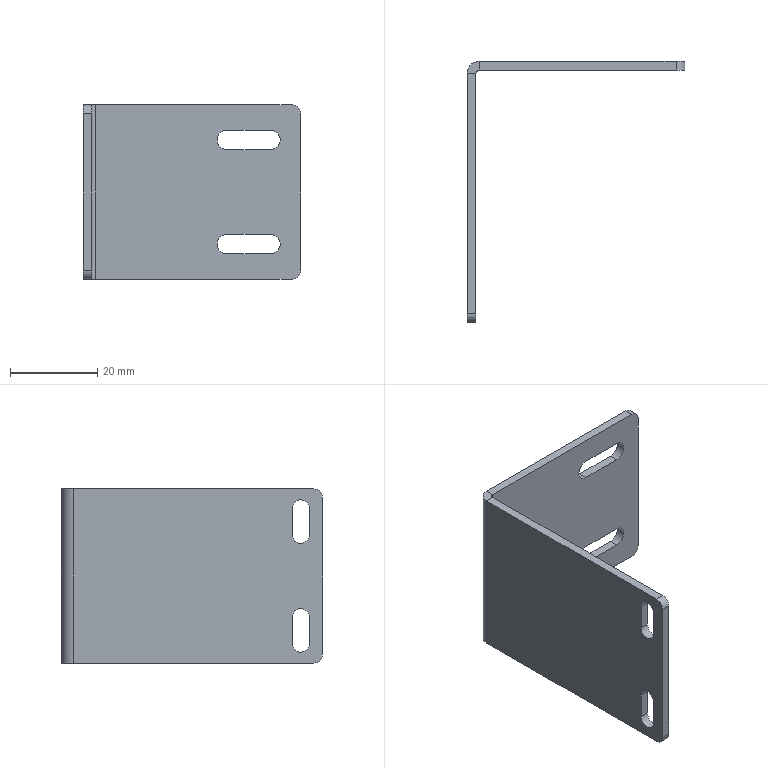Component | SolidWorks | MaterialDetectionSensorMountingPlate-2 | 1 solid | 34 faces | box 50 x 60 x 40 mm | volume 8184 mm3 | plane 20 | cylinder 14 | commonest cylinder face diameters 4 x8 4.5 x4 1.473 x1 5.473 x1
STEP:
#1=COLOUR_RGB('',0.7922,0.8196,0.9333);
#2=FILL_AREA_STYLE_COLOUR('',#1);
#3=FILL_AREA_STYLE('',(#2));
#4=SURFACE_STYLE_FILL_AREA(#3);
#5=SURFACE_SIDE_STYLE('',(#4));
#6=SURFACE_STYLE_USAGE(.BOTH.,#5);
#7=PRESENTATION_STYLE_ASSIGNMENT((#6));
#8=CARTESIAN_POINT('',(-8.239,51.713,4.331));
#9=VERTEX_POINT('',#8);
#10=CARTESIAN_POINT('',(-8.239,51.634,4.331));
#11=VERTEX_POINT('',#10);
#12=CARTESIAN_POINT('',(-8.239,51.713,4.331));
#13=DIRECTION('',(0.,-1.,0.));
#14=VECTOR('',#13,39.37);
#15=LINE('',#12,#14);
#16=EDGE_CURVE('',#9,#11,#15,.T.);
#17=ORIENTED_EDGE('',*,*,#16,.F.);
#18=CARTESIAN_POINT('',(-8.346,51.605,4.331));
#19=VERTEX_POINT('',#18);
#20=CARTESIAN_POINT('',(-8.239,51.605,4.331));
#21=DIRECTION('',(0.,0.,1.));
#22=DIRECTION('',(-1.,0.,0.));
#23=AXIS2_PLACEMENT_3D('',#20,#21,#22);
#24=CIRCLE('',#23,0.1077);
#25=EDGE_CURVE('',#9,#19,#24,.T.);
#26=ORIENTED_EDGE('',*,*,#25,.T.);
#27=CARTESIAN_POINT('',(-8.268,51.605,4.331));
#28=VERTEX_POINT('',#27);
#29=CARTESIAN_POINT('',(-8.268,51.605,4.331));
#30=DIRECTION('',(-1.,-0.,0.));
#31=VECTOR('',#30,39.37);
#32=LINE('',#29,#31);
#33=EDGE_CURVE('',#28,#19,#32,.T.);
#34=ORIENTED_EDGE('',*,*,#33,.F.);
#35=CARTESIAN_POINT('',(-8.239,51.605,4.331));
#36=DIRECTION('',(0.,0.,1.));
#37=DIRECTION('',(1.,0.,0.));
#38=AXIS2_PLACEMENT_3D('',#35,#36,#37);
#39=CIRCLE('',#38,0.029);
#40=EDGE_CURVE('',#11,#28,#39,.T.);
#41=ORIENTED_EDGE('',*,*,#40,.F.);
#42=EDGE_LOOP('',(#17,#26,#34,#41));
#43=FACE_OUTER_BOUND('',#42,.T.);
#44=CARTESIAN_POINT('',(-8.239,51.713,4.331));
#45=DIRECTION('',(0.,0.,1.));
#46=DIRECTION('',(1.,0.,0.));
#47=AXIS2_PLACEMENT_3D('',#44,#45,#46);
#48=PLANE('',#47);
#49=ADVANCED_FACE('',(#43),#48,.T.);
#50=CARTESIAN_POINT('',(-6.457,51.634,4.331));
#51=VERTEX_POINT('',#50);
#52=CARTESIAN_POINT('',(-8.346,51.634,4.331));
#53=DIRECTION('',(-1.,0.,0.));
#54=VECTOR('',#53,39.37);
#55=LINE('',#52,#54);
#56=EDGE_CURVE('',#51,#11,#55,.T.);
#57=ORIENTED_EDGE('',*,*,#56,.F.);
#58=CARTESIAN_POINT('',(-6.457,51.713,4.331));
#59=VERTEX_POINT('',#58);
#60=CARTESIAN_POINT('',(-6.457,51.605,4.331));
#61=DIRECTION('',(0.,1.,0.));
#62=VECTOR('',#61,39.37);
#63=LINE('',#60,#62);
#64=EDGE_CURVE('',#51,#59,#63,.T.);
#65=ORIENTED_EDGE('',*,*,#64,.T.);
#66=CARTESIAN_POINT('',(-8.346,51.713,4.331));
#67=DIRECTION('',(-1.,0.,0.));
#68=VECTOR('',#67,39.37);
#69=LINE('',#66,#68);
#70=EDGE_CURVE('',#59,#9,#69,.T.);
#71=ORIENTED_EDGE('',*,*,#70,.T.);
#72=ORIENTED_EDGE('',*,*,#16,.T.);
#73=EDGE_LOOP('',(#57,#65,#71,#72));
#74=FACE_OUTER_BOUND('',#73,.T.);
#75=CARTESIAN_POINT('',(-8.268,51.605,4.331));
#76=DIRECTION('',(0.,0.,1.));
#77=DIRECTION('',(1.,0.,0.));
#78=AXIS2_PLACEMENT_3D('',#75,#76,#77);
#79=PLANE('',#78);
#80=ADVANCED_FACE('',(#74),#79,.T.);
#81=CARTESIAN_POINT('',(-8.346,51.605,2.756));
#82=VERTEX_POINT('',#81);
#83=CARTESIAN_POINT('',(-8.268,51.605,2.756));
#84=VERTEX_POINT('',#83);
#85=CARTESIAN_POINT('',(-8.346,51.605,2.756));
#86=DIRECTION('',(1.,0.,0.));
#87=VECTOR('',#86,39.37);
#88=LINE('',#85,#87);
#89=EDGE_CURVE('',#82,#84,#88,.T.);
#90=ORIENTED_EDGE('',*,*,#89,.F.);
#91=CARTESIAN_POINT('',(-8.239,51.713,2.756));
#92=VERTEX_POINT('',#91);
#93=CARTESIAN_POINT('',(-8.239,51.605,2.756));
#94=DIRECTION('',(0.,0.,1.));
#95=DIRECTION('',(-1.,0.,0.));
#96=AXIS2_PLACEMENT_3D('',#93,#94,#95);
#97=CIRCLE('',#96,0.1077);
#98=EDGE_CURVE('',#92,#82,#97,.T.);
#99=ORIENTED_EDGE('',*,*,#98,.F.);
#100=CARTESIAN_POINT('',(-8.239,51.634,2.756));
#101=VERTEX_POINT('',#100);
#102=CARTESIAN_POINT('',(-8.239,51.634,2.756));
#103=DIRECTION('',(0.,1.,0.));
#104=VECTOR('',#103,39.37);
#105=LINE('',#102,#104);
#106=EDGE_CURVE('',#101,#92,#105,.T.);
#107=ORIENTED_EDGE('',*,*,#106,.F.);
#108=CARTESIAN_POINT('',(-8.239,51.605,2.756));
#109=DIRECTION('',(0.,0.,1.));
#110=DIRECTION('',(1.,0.,0.));
#111=AXIS2_PLACEMENT_3D('',#108,#109,#110);
#112=CIRCLE('',#111,0.029);
#113=EDGE_CURVE('',#101,#84,#112,.T.);
#114=ORIENTED_EDGE('',*,*,#113,.T.);
#115=EDGE_LOOP('',(#90,#99,#107,#114));
#116=FACE_OUTER_BOUND('',#115,.T.);
#117=CARTESIAN_POINT('',(-8.346,51.605,2.756));
#118=DIRECTION('',(0.,0.,-1.));
#119=DIRECTION('',(-1.,0.,0.));
#120=AXIS2_PLACEMENT_3D('',#117,#118,#119);
#121=PLANE('',#120);
#122=ADVANCED_FACE('',(#116),#121,.T.);
#123=CARTESIAN_POINT('',(-8.268,49.429,2.756));
#124=VERTEX_POINT('',#123);
#125=CARTESIAN_POINT('',(-8.268,51.713,2.756));
#126=DIRECTION('',(0.,-1.,0.));
#127=VECTOR('',#126,39.37);
#128=LINE('',#125,#127);
#129=EDGE_CURVE('',#84,#124,#128,.T.);
#130=ORIENTED_EDGE('',*,*,#129,.T.);
#131=CARTESIAN_POINT('',(-8.346,49.429,2.756));
#132=VERTEX_POINT('',#131);
#133=CARTESIAN_POINT('',(-8.239,49.429,2.756));
#134=DIRECTION('',(-1.,0.,0.));
#135=VECTOR('',#134,39.37);
#136=LINE('',#133,#135);
#137=EDGE_CURVE('',#124,#132,#136,.T.);
#138=ORIENTED_EDGE('',*,*,#137,.T.);
#139=CARTESIAN_POINT('',(-8.346,51.713,2.756));
#140=DIRECTION('',(0.,-1.,0.));
#141=VECTOR('',#140,39.37);
#142=LINE('',#139,#141);
#143=EDGE_CURVE('',#82,#132,#142,.T.);
#144=ORIENTED_EDGE('',*,*,#143,.F.);
#145=ORIENTED_EDGE('',*,*,#89,.T.);
#146=EDGE_LOOP('',(#130,#138,#144,#145));
#147=FACE_OUTER_BOUND('',#146,.T.);
#148=CARTESIAN_POINT('',(-8.239,51.634,2.756));
#149=DIRECTION('',(0.,0.,-1.));
#150=DIRECTION('',(-1.,0.,0.));
#151=AXIS2_PLACEMENT_3D('',#148,#149,#150);
#152=PLANE('',#151);
#153=ADVANCED_FACE('',(#147),#152,.T.);
#154=CARTESIAN_POINT('',(-8.346,49.469,3.917));
#155=VERTEX_POINT('',#154);
#156=CARTESIAN_POINT('',(-8.346,49.469,4.154));
#157=VERTEX_POINT('',#156);
#158=CARTESIAN_POINT('',(-8.346,49.469,3.917));
#159=DIRECTION('',(0.,0.,1.));
#160=VECTOR('',#159,39.37);
#161=LINE('',#158,#160);
#162=EDGE_CURVE('',#155,#157,#161,.T.);
#163=ORIENTED_EDGE('',*,*,#162,.F.);
#164=CARTESIAN_POINT('',(-8.346,49.626,3.917));
#165=VERTEX_POINT('',#164);
#166=CARTESIAN_POINT('',(-8.346,49.547,3.917));
#167=DIRECTION('',(-1.,-0.,0.));
#168=DIRECTION('',(0.,-1.,0.));
#169=AXIS2_PLACEMENT_3D('',#166,#167,#168);
#170=CIRCLE('',#169,0.07874);
#171=EDGE_CURVE('',#165,#155,#170,.T.);
#172=ORIENTED_EDGE('',*,*,#171,.F.);
#173=CARTESIAN_POINT('',(-8.346,49.626,4.154));
#174=VERTEX_POINT('',#173);
#175=CARTESIAN_POINT('',(-8.346,49.626,3.917));
#176=DIRECTION('',(0.,0.,-1.));
#177=VECTOR('',#176,39.37);
#178=LINE('',#175,#177);
#179=EDGE_CURVE('',#174,#165,#178,.T.);
#180=ORIENTED_EDGE('',*,*,#179,.F.);
#181=CARTESIAN_POINT('',(-8.346,49.547,4.154));
#182=DIRECTION('',(-1.,-0.,0.));
#183=DIRECTION('',(0.,-1.,0.));
#184=AXIS2_PLACEMENT_3D('',#181,#182,#183);
#185=CIRCLE('',#184,0.07874);
#186=EDGE_CURVE('',#157,#174,#185,.T.);
#187=ORIENTED_EDGE('',*,*,#186,.F.);
#188=EDGE_LOOP('',(#163,#172,#180,#187));
#189=FACE_BOUND('',#188,.T.);
#190=CARTESIAN_POINT('',(-8.346,49.469,2.933));
#191=VERTEX_POINT('',#190);
#192=CARTESIAN_POINT('',(-8.346,49.469,3.169));
#193=VERTEX_POINT('',#192);
#194=CARTESIAN_POINT('',(-8.346,49.469,2.933));
#195=DIRECTION('',(0.,0.,1.));
#196=VECTOR('',#195,39.37);
#197=LINE('',#194,#196);
#198=EDGE_CURVE('',#191,#193,#197,.T.);
#199=ORIENTED_EDGE('',*,*,#198,.F.);
#200=CARTESIAN_POINT('',(-8.346,49.626,2.933));
#201=VERTEX_POINT('',#200);
#202=CARTESIAN_POINT('',(-8.346,49.547,2.933));
#203=DIRECTION('',(-1.,-0.,0.));
#204=DIRECTION('',(0.,-1.,0.));
#205=AXIS2_PLACEMENT_3D('',#202,#203,#204);
#206=CIRCLE('',#205,0.07874);
#207=EDGE_CURVE('',#201,#191,#206,.T.);
#208=ORIENTED_EDGE('',*,*,#207,.F.);
#209=CARTESIAN_POINT('',(-8.346,49.626,3.169));
#210=VERTEX_POINT('',#209);
#211=CARTESIAN_POINT('',(-8.346,49.626,2.933));
#212=DIRECTION('',(0.,0.,-1.));
#213=VECTOR('',#212,39.37);
#214=LINE('',#211,#213);
#215=EDGE_CURVE('',#210,#201,#214,.T.);
#216=ORIENTED_EDGE('',*,*,#215,.F.);
#217=CARTESIAN_POINT('',(-8.346,49.547,3.169));
#218=DIRECTION('',(-1.,-0.,0.));
#219=DIRECTION('',(0.,-1.,0.));
#220=AXIS2_PLACEMENT_3D('',#217,#218,#219);
#221=CIRCLE('',#220,0.07874);
#222=EDGE_CURVE('',#193,#210,#221,.T.);
#223=ORIENTED_EDGE('',*,*,#222,.F.);
#224=EDGE_LOOP('',(#199,#208,#216,#223));
#225=FACE_BOUND('',#224,.T.);
#226=CARTESIAN_POINT('',(-8.346,49.35,4.252));
#227=VERTEX_POINT('',#226);
#228=CARTESIAN_POINT('',(-8.346,49.35,2.835));
#229=VERTEX_POINT('',#228);
#230=CARTESIAN_POINT('',(-8.346,49.35,4.331));
#231=DIRECTION('',(0.,0.,-1.));
#232=VECTOR('',#231,39.37);
#233=LINE('',#230,#232);
#234=EDGE_CURVE('',#227,#229,#233,.T.);
#235=ORIENTED_EDGE('',*,*,#234,.F.);
#236=CARTESIAN_POINT('',(-8.346,49.429,4.331));
#237=VERTEX_POINT('',#236);
#238=CARTESIAN_POINT('',(-8.346,49.429,4.252));
#239=DIRECTION('',(-1.,-0.,0.));
#240=DIRECTION('',(0.,1.,0.));
#241=AXIS2_PLACEMENT_3D('',#238,#239,#240);
#242=CIRCLE('',#241,0.07874);
#243=EDGE_CURVE('',#227,#237,#242,.T.);
#244=ORIENTED_EDGE('',*,*,#243,.T.);
#245=CARTESIAN_POINT('',(-8.346,51.713,4.331));
#246=DIRECTION('',(0.,-1.,0.));
#247=VECTOR('',#246,39.37);
#248=LINE('',#245,#247);
#249=EDGE_CURVE('',#19,#237,#248,.T.);
#250=ORIENTED_EDGE('',*,*,#249,.F.);
#251=CARTESIAN_POINT('',(-8.346,51.605,4.331));
#252=DIRECTION('',(0.,0.,-1.));
#253=VECTOR('',#252,39.37);
#254=LINE('',#251,#253);
#255=EDGE_CURVE('',#19,#82,#254,.T.);
#256=ORIENTED_EDGE('',*,*,#255,.T.);
#257=ORIENTED_EDGE('',*,*,#143,.T.);
#258=CARTESIAN_POINT('',(-8.346,49.429,2.835));
#259=DIRECTION('',(-1.,-0.,0.));
#260=DIRECTION('',(0.,1.,0.));
#261=AXIS2_PLACEMENT_3D('',#258,#259,#260);
#262=CIRCLE('',#261,0.07874);
#263=EDGE_CURVE('',#132,#229,#262,.T.);
#264=ORIENTED_EDGE('',*,*,#263,.T.);
#265=EDGE_LOOP('',(#235,#244,#250,#256,#257,#264));
#266=FACE_OUTER_BOUND('',#265,.T.);
#267=CARTESIAN_POINT('',(-8.346,51.713,4.331));
#268=DIRECTION('',(1.,0.,0.));
#269=DIRECTION('',(-0.,1.,0.));
#270=AXIS2_PLACEMENT_3D('',#267,#268,#269);
#271=PLANE('',#270);
#272=ADVANCED_FACE('',(#189,#225,#266),#271,.F.);
#273=CARTESIAN_POINT('',(-8.268,49.35,4.252));
#274=VERTEX_POINT('',#273);
#275=CARTESIAN_POINT('',(-8.268,49.35,2.835));
#276=VERTEX_POINT('',#275);
#277=CARTESIAN_POINT('',(-8.268,49.35,4.331));
#278=DIRECTION('',(0.,0.,-1.));
#279=VECTOR('',#278,39.37);
#280=LINE('',#277,#279);
#281=EDGE_CURVE('',#274,#276,#280,.T.);
#282=ORIENTED_EDGE('',*,*,#281,.F.);
#283=CARTESIAN_POINT('',(-8.268,49.35,4.252));
#284=DIRECTION('',(-1.,0.,0.));
#285=VECTOR('',#284,39.37);
#286=LINE('',#283,#285);
#287=EDGE_CURVE('',#274,#227,#286,.T.);
#288=ORIENTED_EDGE('',*,*,#287,.T.);
#289=ORIENTED_EDGE('',*,*,#234,.T.);
#290=CARTESIAN_POINT('',(-8.268,49.35,2.835));
#291=DIRECTION('',(1.,0.,0.));
#292=VECTOR('',#291,39.37);
#293=LINE('',#290,#292);
#294=EDGE_CURVE('',#229,#276,#293,.T.);
#295=ORIENTED_EDGE('',*,*,#294,.T.);
#296=EDGE_LOOP('',(#282,#288,#289,#295));
#297=FACE_OUTER_BOUND('',#296,.T.);
#298=CARTESIAN_POINT('',(-8.268,49.35,4.331));
#299=DIRECTION('',(0.,-1.,0.));
#300=DIRECTION('',(0.,0.,-1.));
#301=AXIS2_PLACEMENT_3D('',#298,#299,#300);
#302=PLANE('',#301);
#303=ADVANCED_FACE('',(#297),#302,.T.);
#304=CARTESIAN_POINT('',(-8.268,49.469,3.917));
#305=VERTEX_POINT('',#304);
#306=CARTESIAN_POINT('',(-8.268,49.626,3.917));
#307=VERTEX_POINT('',#306);
#308=CARTESIAN_POINT('',(-8.268,49.547,3.917));
#309=DIRECTION('',(1.,0.,0.));
#310=DIRECTION('',(0.,1.,0.));
#311=AXIS2_PLACEMENT_3D('',#308,#309,#310);
#312=CIRCLE('',#311,0.07874);
#313=EDGE_CURVE('',#305,#307,#312,.T.);
#314=ORIENTED_EDGE('',*,*,#313,.F.);
#315=CARTESIAN_POINT('',(-8.268,49.469,4.154));
#316=VERTEX_POINT('',#315);
#317=CARTESIAN_POINT('',(-8.268,49.469,4.331));
#318=DIRECTION('',(0.,0.,-1.));
#319=VECTOR('',#318,39.37);
#320=LINE('',#317,#319);
#321=EDGE_CURVE('',#316,#305,#320,.T.);
#322=ORIENTED_EDGE('',*,*,#321,.F.);
#323=CARTESIAN_POINT('',(-8.268,49.626,4.154));
#324=VERTEX_POINT('',#323);
#325=CARTESIAN_POINT('',(-8.268,49.547,4.154));
#326=DIRECTION('',(1.,0.,0.));
#327=DIRECTION('',(0.,1.,0.));
#328=AXIS2_PLACEMENT_3D('',#325,#326,#327);
#329=CIRCLE('',#328,0.07874);
#330=EDGE_CURVE('',#324,#316,#329,.T.);
#331=ORIENTED_EDGE('',*,*,#330,.F.);
#332=CARTESIAN_POINT('',(-8.268,49.626,4.331));
#333=DIRECTION('',(0.,0.,1.));
#334=VECTOR('',#333,39.37);
#335=LINE('',#332,#334);
#336=EDGE_CURVE('',#307,#324,#335,.T.);
#337=ORIENTED_EDGE('',*,*,#336,.F.);
#338=EDGE_LOOP('',(#314,#322,#331,#337));
#339=FACE_BOUND('',#338,.T.);
#340=CARTESIAN_POINT('',(-8.268,49.469,2.933));
#341=VERTEX_POINT('',#340);
#342=CARTESIAN_POINT('',(-8.268,49.626,2.933));
#343=VERTEX_POINT('',#342);
#344=CARTESIAN_POINT('',(-8.268,49.547,2.933));
#345=DIRECTION('',(1.,0.,0.));
#346=DIRECTION('',(0.,1.,0.));
#347=AXIS2_PLACEMENT_3D('',#344,#345,#346);
#348=CIRCLE('',#347,0.07874);
#349=EDGE_CURVE('',#341,#343,#348,.T.);
#350=ORIENTED_EDGE('',*,*,#349,.F.);
#351=CARTESIAN_POINT('',(-8.268,49.469,3.169));
#352=VERTEX_POINT('',#351);
#353=CARTESIAN_POINT('',(-8.268,49.469,4.331));
#354=DIRECTION('',(0.,0.,-1.));
#355=VECTOR('',#354,39.37);
#356=LINE('',#353,#355);
#357=EDGE_CURVE('',#352,#341,#356,.T.);
#358=ORIENTED_EDGE('',*,*,#357,.F.);
#359=CARTESIAN_POINT('',(-8.268,49.626,3.169));
#360=VERTEX_POINT('',#359);
#361=CARTESIAN_POINT('',(-8.268,49.547,3.169));
#362=DIRECTION('',(1.,0.,0.));
#363=DIRECTION('',(0.,1.,0.));
#364=AXIS2_PLACEMENT_3D('',#361,#362,#363);
#365=CIRCLE('',#364,0.07874);
#366=EDGE_CURVE('',#360,#352,#365,.T.);
#367=ORIENTED_EDGE('',*,*,#366,.F.);
#368=CARTESIAN_POINT('',(-8.268,49.626,4.331));
#369=DIRECTION('',(0.,0.,1.));
#370=VECTOR('',#369,39.37);
#371=LINE('',#368,#370);
#372=EDGE_CURVE('',#343,#360,#371,.T.);
#373=ORIENTED_EDGE('',*,*,#372,.F.);
#374=EDGE_LOOP('',(#350,#358,#367,#373));
#375=FACE_BOUND('',#374,.T.);
#376=CARTESIAN_POINT('',(-8.268,49.429,4.331));
#377=VERTEX_POINT('',#376);
#378=CARTESIAN_POINT('',(-8.268,51.713,4.331));
#379=DIRECTION('',(0.,-1.,0.));
#380=VECTOR('',#379,39.37);
#381=LINE('',#378,#380);
#382=EDGE_CURVE('',#28,#377,#381,.T.);
#383=ORIENTED_EDGE('',*,*,#382,.T.);
#384=CARTESIAN_POINT('',(-8.268,49.429,4.252));
#385=DIRECTION('',(1.,0.,0.));
#386=DIRECTION('',(0.,1.,0.));
#387=AXIS2_PLACEMENT_3D('',#384,#385,#386);
#388=CIRCLE('',#387,0.07874);
#389=EDGE_CURVE('',#377,#274,#388,.T.);
#390=ORIENTED_EDGE('',*,*,#389,.T.);
#391=ORIENTED_EDGE('',*,*,#281,.T.);
#392=CARTESIAN_POINT('',(-8.268,49.429,2.835));
#393=DIRECTION('',(1.,0.,0.));
#394=DIRECTION('',(0.,1.,0.));
#395=AXIS2_PLACEMENT_3D('',#392,#393,#394);
#396=CIRCLE('',#395,0.07874);
#397=EDGE_CURVE('',#276,#124,#396,.T.);
#398=ORIENTED_EDGE('',*,*,#397,.T.);
#399=ORIENTED_EDGE('',*,*,#129,.F.);
#400=CARTESIAN_POINT('',(-8.268,51.605,4.331));
#401=DIRECTION('',(0.,0.,-1.));
#402=VECTOR('',#401,39.37);
#403=LINE('',#400,#402);
#404=EDGE_CURVE('',#28,#84,#403,.T.);
#405=ORIENTED_EDGE('',*,*,#404,.F.);
#406=EDGE_LOOP('',(#383,#390,#391,#398,#399,#405));
#407=FACE_OUTER_BOUND('',#406,.T.);
#408=CARTESIAN_POINT('',(-8.268,51.713,4.331));
#409=DIRECTION('',(1.,0.,0.));
#410=DIRECTION('',(-0.,1.,0.));
#411=AXIS2_PLACEMENT_3D('',#408,#409,#410);
#412=PLANE('',#411);
#413=ADVANCED_FACE('',(#339,#375,#407),#412,.T.);
#414=ORIENTED_EDGE('',*,*,#113,.F.);
#415=CARTESIAN_POINT('',(-8.239,51.634,4.331));
#416=DIRECTION('',(0.,0.,-1.));
#417=VECTOR('',#416,39.37);
#418=LINE('',#415,#417);
#419=EDGE_CURVE('',#11,#101,#418,.T.);
#420=ORIENTED_EDGE('',*,*,#419,.F.);
#421=ORIENTED_EDGE('',*,*,#40,.T.);
#422=ORIENTED_EDGE('',*,*,#404,.T.);
#423=EDGE_LOOP('',(#414,#420,#421,#422));
#424=FACE_OUTER_BOUND('',#423,.T.);
#425=CARTESIAN_POINT('',(-8.239,51.605,4.331));
#426=DIRECTION('',(0.,0.,-1.));
#427=DIRECTION('',(-1.,0.,0.));
#428=AXIS2_PLACEMENT_3D('',#425,#426,#427);
#429=CYLINDRICAL_SURFACE('',#428,0.029);
#430=ADVANCED_FACE('',(#424),#429,.F.);
#431=CARTESIAN_POINT('',(-7.047,51.634,4.104));
#432=VERTEX_POINT('',#431);
#433=CARTESIAN_POINT('',(-7.047,51.634,3.927));
#434=VERTEX_POINT('',#433);
#435=CARTESIAN_POINT('',(-7.047,51.634,4.016));
#436=DIRECTION('',(0.,-1.,0.));
#437=DIRECTION('',(0.,0.,-1.));
#438=AXIS2_PLACEMENT_3D('',#435,#436,#437);
#439=CIRCLE('',#438,0.08858);
#440=EDGE_CURVE('',#432,#434,#439,.T.);
#441=ORIENTED_EDGE('',*,*,#440,.F.);
#442=CARTESIAN_POINT('',(-6.654,51.634,4.104));
#443=VERTEX_POINT('',#442);
#444=CARTESIAN_POINT('',(-8.346,51.634,4.104));
#445=DIRECTION('',(-1.,0.,0.));
#446=VECTOR('',#445,39.37);
#447=LINE('',#444,#446);
#448=EDGE_CURVE('',#443,#432,#447,.T.);
#449=ORIENTED_EDGE('',*,*,#448,.F.);
#450=CARTESIAN_POINT('',(-6.654,51.634,3.927));
#451=VERTEX_POINT('',#450);
#452=CARTESIAN_POINT('',(-6.654,51.634,4.016));
#453=DIRECTION('',(0.,-1.,0.));
#454=DIRECTION('',(0.,0.,-1.));
#455=AXIS2_PLACEMENT_3D('',#452,#453,#454);
#456=CIRCLE('',#455,0.08858);
#457=EDGE_CURVE('',#451,#443,#456,.T.);
#458=ORIENTED_EDGE('',*,*,#457,.F.);
#459=CARTESIAN_POINT('',(-8.346,51.634,3.927));
#460=DIRECTION('',(1.,0.,0.));
#461=VECTOR('',#460,39.37);
#462=LINE('',#459,#461);
#463=EDGE_CURVE('',#434,#451,#462,.T.);
#464=ORIENTED_EDGE('',*,*,#463,.F.);
#465=EDGE_LOOP('',(#441,#449,#458,#464));
#466=FACE_BOUND('',#465,.T.);
#467=CARTESIAN_POINT('',(-7.047,51.634,3.159));
#468=VERTEX_POINT('',#467);
#469=CARTESIAN_POINT('',(-7.047,51.634,2.982));
#470=VERTEX_POINT('',#469);
#471=CARTESIAN_POINT('',(-7.047,51.634,3.071));
#472=DIRECTION('',(0.,-1.,0.));
#473=DIRECTION('',(0.,0.,-1.));
#474=AXIS2_PLACEMENT_3D('',#471,#472,#473);
#475=CIRCLE('',#474,0.08858);
#476=EDGE_CURVE('',#468,#470,#475,.T.);
#477=ORIENTED_EDGE('',*,*,#476,.F.);
#478=CARTESIAN_POINT('',(-6.654,51.634,3.159));
#479=VERTEX_POINT('',#478);
#480=CARTESIAN_POINT('',(-8.346,51.634,3.159));
#481=DIRECTION('',(-1.,0.,0.));
#482=VECTOR('',#481,39.37);
#483=LINE('',#480,#482);
#484=EDGE_CURVE('',#479,#468,#483,.T.);
#485=ORIENTED_EDGE('',*,*,#484,.F.);
#486=CARTESIAN_POINT('',(-6.654,51.634,2.982));
#487=VERTEX_POINT('',#486);
#488=CARTESIAN_POINT('',(-6.654,51.634,3.071));
#489=DIRECTION('',(0.,-1.,0.));
#490=DIRECTION('',(0.,0.,-1.));
#491=AXIS2_PLACEMENT_3D('',#488,#489,#490);
#492=CIRCLE('',#491,0.08858);
#493=EDGE_CURVE('',#487,#479,#492,.T.);
#494=ORIENTED_EDGE('',*,*,#493,.F.);
#495=CARTESIAN_POINT('',(-8.346,51.634,2.982));
#496=DIRECTION('',(1.,0.,0.));
#497=VECTOR('',#496,39.37);
#498=LINE('',#495,#497);
#499=EDGE_CURVE('',#470,#487,#498,.T.);
#500=ORIENTED_EDGE('',*,*,#499,.F.);
#501=EDGE_LOOP('',(#477,#485,#494,#500));
#502=FACE_BOUND('',#501,.T.);
#503=CARTESIAN_POINT('',(-6.457,51.634,2.756));
#504=VERTEX_POINT('',#503);
#505=CARTESIAN_POINT('',(-8.346,51.634,2.756));
#506=DIRECTION('',(-1.,0.,0.));
#507=VECTOR('',#506,39.37);
#508=LINE('',#505,#507);
#509=EDGE_CURVE('',#504,#101,#508,.T.);
#510=ORIENTED_EDGE('',*,*,#509,.F.);
#511=CARTESIAN_POINT('',(-6.378,51.634,2.835));
#512=VERTEX_POINT('',#511);
#513=CARTESIAN_POINT('',(-6.457,51.634,2.835));
#514=DIRECTION('',(0.,-1.,0.));
#515=DIRECTION('',(0.,0.,-1.));
#516=AXIS2_PLACEMENT_3D('',#513,#514,#515);
#517=CIRCLE('',#516,0.07874);
#518=EDGE_CURVE('',#504,#512,#517,.T.);
#519=ORIENTED_EDGE('',*,*,#518,.T.);
#520=CARTESIAN_POINT('',(-6.378,51.634,4.252));
#521=VERTEX_POINT('',#520);
#522=CARTESIAN_POINT('',(-6.378,51.634,4.331));
#523=DIRECTION('',(0.,0.,-1.));
#524=VECTOR('',#523,39.37);
#525=LINE('',#522,#524);
#526=EDGE_CURVE('',#521,#512,#525,.T.);
#527=ORIENTED_EDGE('',*,*,#526,.F.);
#528=CARTESIAN_POINT('',(-6.457,51.634,4.252));
#529=DIRECTION('',(0.,-1.,0.));
#530=DIRECTION('',(0.,0.,-1.));
#531=AXIS2_PLACEMENT_3D('',#528,#529,#530);
#532=CIRCLE('',#531,0.07874);
#533=EDGE_CURVE('',#521,#51,#532,.T.);
#534=ORIENTED_EDGE('',*,*,#533,.T.);
#535=ORIENTED_EDGE('',*,*,#56,.T.);
#536=ORIENTED_EDGE('',*,*,#419,.T.);
#537=EDGE_LOOP('',(#510,#519,#527,#534,#535,#536));
#538=FACE_OUTER_BOUND('',#537,.T.);
#539=CARTESIAN_POINT('',(-8.346,51.634,4.331));
#540=DIRECTION('',(0.,-1.,0.));
#541=DIRECTION('',(0.,0.,-1.));
#542=AXIS2_PLACEMENT_3D('',#539,#540,#541);
#543=PLANE('',#542);
#544=ADVANCED_FACE('',(#466,#502,#538),#543,.T.);
#545=ORIENTED_EDGE('',*,*,#526,.T.);
#546=CARTESIAN_POINT('',(-6.378,51.713,2.835));
#547=VERTEX_POINT('',#546);
#548=CARTESIAN_POINT('',(-6.378,51.713,2.835));
#549=DIRECTION('',(0.,1.,0.));
#550=VECTOR('',#549,39.37);
#551=LINE('',#548,#550);
#552=EDGE_CURVE('',#512,#547,#551,.T.);
#553=ORIENTED_EDGE('',*,*,#552,.T.);
#554=CARTESIAN_POINT('',(-6.378,51.713,4.252));
#555=VERTEX_POINT('',#554);
#556=CARTESIAN_POINT('',(-6.378,51.713,4.331));
#557=DIRECTION('',(0.,0.,-1.));
#558=VECTOR('',#557,39.37);
#559=LINE('',#556,#558);
#560=EDGE_CURVE('',#555,#547,#559,.T.);
#561=ORIENTED_EDGE('',*,*,#560,.F.);
#562=CARTESIAN_POINT('',(-6.378,51.713,4.252));
#563=DIRECTION('',(0.,-1.,0.));
#564=VECTOR('',#563,39.37);
#565=LINE('',#562,#564);
#566=EDGE_CURVE('',#555,#521,#565,.T.);
#567=ORIENTED_EDGE('',*,*,#566,.T.);
#568=EDGE_LOOP('',(#545,#553,#561,#567));
#569=FACE_OUTER_BOUND('',#568,.T.);
#570=CARTESIAN_POINT('',(-6.378,51.713,4.331));
#571=DIRECTION('',(1.,0.,0.));
#572=DIRECTION('',(0.,0.,-1.));
#573=AXIS2_PLACEMENT_3D('',#570,#571,#572);
#574=PLANE('',#573);
#575=ADVANCED_FACE('',(#569),#574,.T.);
#576=CARTESIAN_POINT('',(-7.047,51.713,4.104));
#577=VERTEX_POINT('',#576);
#578=CARTESIAN_POINT('',(-6.654,51.713,4.104));
#579=VERTEX_POINT('',#578);
#580=CARTESIAN_POINT('',(-7.047,51.713,4.104));
#581=DIRECTION('',(1.,0.,0.));
#582=VECTOR('',#581,39.37);
#583=LINE('',#580,#582);
#584=EDGE_CURVE('',#577,#579,#583,.T.);
#585=ORIENTED_EDGE('',*,*,#584,.F.);
#586=CARTESIAN_POINT('',(-7.047,51.713,3.927));
#587=VERTEX_POINT('',#586);
#588=CARTESIAN_POINT('',(-7.047,51.713,4.016));
#589=DIRECTION('',(0.,1.,0.));
#590=DIRECTION('',(0.,0.,1.));
#591=AXIS2_PLACEMENT_3D('',#588,#589,#590);
#592=CIRCLE('',#591,0.08858);
#593=EDGE_CURVE('',#587,#577,#592,.T.);
#594=ORIENTED_EDGE('',*,*,#593,.F.);
#595=CARTESIAN_POINT('',(-6.654,51.713,3.927));
#596=VERTEX_POINT('',#595);
#597=CARTESIAN_POINT('',(-7.047,51.713,3.927));
#598=DIRECTION('',(-1.,0.,0.));
#599=VECTOR('',#598,39.37);
#600=LINE('',#597,#599);
#601=EDGE_CURVE('',#596,#587,#600,.T.);
#602=ORIENTED_EDGE('',*,*,#601,.F.);
#603=CARTESIAN_POINT('',(-6.654,51.713,4.016));
#604=DIRECTION('',(0.,1.,0.));
#605=DIRECTION('',(0.,0.,1.));
#606=AXIS2_PLACEMENT_3D('',#603,#604,#605);
#607=CIRCLE('',#606,0.08858);
#608=EDGE_CURVE('',#579,#596,#607,.T.);
#609=ORIENTED_EDGE('',*,*,#608,.F.);
#610=EDGE_LOOP('',(#585,#594,#602,#609));
#611=FACE_BOUND('',#610,.T.);
#612=CARTESIAN_POINT('',(-7.047,51.713,3.159));
#613=VERTEX_POINT('',#612);
#614=CARTESIAN_POINT('',(-6.654,51.713,3.159));
#615=VERTEX_POINT('',#614);
#616=CARTESIAN_POINT('',(-7.047,51.713,3.159));
#617=DIRECTION('',(1.,0.,0.));
#618=VECTOR('',#617,39.37);
#619=LINE('',#616,#618);
#620=EDGE_CURVE('',#613,#615,#619,.T.);
#621=ORIENTED_EDGE('',*,*,#620,.F.);
#622=CARTESIAN_POINT('',(-7.047,51.713,2.982));
#623=VERTEX_POINT('',#622);
#624=CARTESIAN_POINT('',(-7.047,51.713,3.071));
#625=DIRECTION('',(0.,1.,0.));
#626=DIRECTION('',(0.,0.,1.));
#627=AXIS2_PLACEMENT_3D('',#624,#625,#626);
#628=CIRCLE('',#627,0.08858);
#629=EDGE_CURVE('',#623,#613,#628,.T.);
#630=ORIENTED_EDGE('',*,*,#629,.F.);
#631=CARTESIAN_POINT('',(-6.654,51.713,2.982));
#632=VERTEX_POINT('',#631);
#633=CARTESIAN_POINT('',(-7.047,51.713,2.982));
#634=DIRECTION('',(-1.,0.,0.));
#635=VECTOR('',#634,39.37);
#636=LINE('',#633,#635);
#637=EDGE_CURVE('',#632,#623,#636,.T.);
#638=ORIENTED_EDGE('',*,*,#637,.F.);
#639=CARTESIAN_POINT('',(-6.654,51.713,3.071));
#640=DIRECTION('',(0.,1.,0.));
#641=DIRECTION('',(0.,0.,1.));
#642=AXIS2_PLACEMENT_3D('',#639,#640,#641);
#643=CIRCLE('',#642,0.08858);
#644=EDGE_CURVE('',#615,#632,#643,.T.);
#645=ORIENTED_EDGE('',*,*,#644,.F.);
#646=EDGE_LOOP('',(#621,#630,#638,#645));
#647=FACE_BOUND('',#646,.T.);
#648=ORIENTED_EDGE('',*,*,#560,.T.);
#649=CARTESIAN_POINT('',(-6.457,51.713,2.756));
#650=VERTEX_POINT('',#649);
#651=CARTESIAN_POINT('',(-6.457,51.713,2.835));
#652=DIRECTION('',(0.,1.,0.));
#653=DIRECTION('',(0.,0.,-1.));
#654=AXIS2_PLACEMENT_3D('',#651,#652,#653);
#655=CIRCLE('',#654,0.07874);
#656=EDGE_CURVE('',#547,#650,#655,.T.);
#657=ORIENTED_EDGE('',*,*,#656,.T.);
#658=CARTESIAN_POINT('',(-8.346,51.713,2.756));
#659=DIRECTION('',(-1.,0.,0.));
#660=VECTOR('',#659,39.37);
#661=LINE('',#658,#660);
#662=EDGE_CURVE('',#650,#92,#661,.T.);
#663=ORIENTED_EDGE('',*,*,#662,.T.);
#664=CARTESIAN_POINT('',(-8.239,51.713,4.331));
#665=DIRECTION('',(0.,0.,-1.));
#666=VECTOR('',#665,39.37);
#667=LINE('',#664,#666);
#668=EDGE_CURVE('',#9,#92,#667,.T.);
#669=ORIENTED_EDGE('',*,*,#668,.F.);
#670=ORIENTED_EDGE('',*,*,#70,.F.);
#671=CARTESIAN_POINT('',(-6.457,51.713,4.252));
#672=DIRECTION('',(0.,1.,0.));
#673=DIRECTION('',(0.,0.,-1.));
#674=AXIS2_PLACEMENT_3D('',#671,#672,#673);
#675=CIRCLE('',#674,0.07874);
#676=EDGE_CURVE('',#59,#555,#675,.T.);
#677=ORIENTED_EDGE('',*,*,#676,.T.);
#678=EDGE_LOOP('',(#648,#657,#663,#669,#670,#677));
#679=FACE_OUTER_BOUND('',#678,.T.);
#680=CARTESIAN_POINT('',(-8.346,51.713,4.331));
#681=DIRECTION('',(0.,-1.,0.));
#682=DIRECTION('',(0.,0.,-1.));
#683=AXIS2_PLACEMENT_3D('',#680,#681,#682);
#684=PLANE('',#683);
#685=ADVANCED_FACE('',(#611,#647,#679),#684,.F.);
#686=ORIENTED_EDGE('',*,*,#98,.T.);
#687=ORIENTED_EDGE('',*,*,#255,.F.);
#688=ORIENTED_EDGE('',*,*,#25,.F.);
#689=ORIENTED_EDGE('',*,*,#668,.T.);
#690=EDGE_LOOP('',(#686,#687,#688,#689));
#691=FACE_OUTER_BOUND('',#690,.T.);
#692=CARTESIAN_POINT('',(-8.239,51.605,4.331));
#693=DIRECTION('',(0.,0.,-1.));
#694=DIRECTION('',(-1.,0.,0.));
#695=AXIS2_PLACEMENT_3D('',#692,#693,#694);
#696=CYLINDRICAL_SURFACE('',#695,0.1077);
#697=ADVANCED_FACE('',(#691),#696,.T.);
#698=ORIENTED_EDGE('',*,*,#249,.T.);
#699=CARTESIAN_POINT('',(-8.239,49.429,4.331));
#700=DIRECTION('',(1.,0.,0.));
#701=VECTOR('',#700,39.37);
#702=LINE('',#699,#701);
#703=EDGE_CURVE('',#237,#377,#702,.T.);
#704=ORIENTED_EDGE('',*,*,#703,.T.);
#705=ORIENTED_EDGE('',*,*,#382,.F.);
#706=ORIENTED_EDGE('',*,*,#33,.T.);
#707=EDGE_LOOP('',(#698,#704,#705,#706));
#708=FACE_OUTER_BOUND('',#707,.T.);
#709=CARTESIAN_POINT('',(-8.239,51.605,4.331));
#710=DIRECTION('',(0.,0.,1.));
#711=DIRECTION('',(1.,0.,0.));
#712=AXIS2_PLACEMENT_3D('',#709,#710,#711);
#713=PLANE('',#712);
#714=ADVANCED_FACE('',(#708),#713,.T.);
#715=ORIENTED_EDGE('',*,*,#662,.F.);
#716=CARTESIAN_POINT('',(-6.457,51.634,2.756));
#717=DIRECTION('',(0.,-1.,0.));
#718=VECTOR('',#717,39.37);
#719=LINE('',#716,#718);
#720=EDGE_CURVE('',#650,#504,#719,.T.);
#721=ORIENTED_EDGE('',*,*,#720,.T.);
#722=ORIENTED_EDGE('',*,*,#509,.T.);
#723=ORIENTED_EDGE('',*,*,#106,.T.);
#724=EDGE_LOOP('',(#715,#721,#722,#723));
#725=FACE_OUTER_BOUND('',#724,.T.);
#726=CARTESIAN_POINT('',(-8.239,51.605,2.756));
#727=DIRECTION('',(0.,0.,1.));
#728=DIRECTION('',(1.,0.,0.));
#729=AXIS2_PLACEMENT_3D('',#726,#727,#728);
#730=PLANE('',#729);
#731=ADVANCED_FACE('',(#725),#730,.F.);
#732=ORIENTED_EDGE('',*,*,#389,.F.);
#733=ORIENTED_EDGE('',*,*,#703,.F.);
#734=ORIENTED_EDGE('',*,*,#243,.F.);
#735=ORIENTED_EDGE('',*,*,#287,.F.);
#736=EDGE_LOOP('',(#732,#733,#734,#735));
#737=FACE_OUTER_BOUND('',#736,.T.);
#738=CARTESIAN_POINT('',(-8.268,49.429,4.252));
#739=DIRECTION('',(-1.,0.,0.));
#740=DIRECTION('',(0.,0.,1.));
#741=AXIS2_PLACEMENT_3D('',#738,#739,#740);
#742=CYLINDRICAL_SURFACE('',#741,0.07874);
#743=ADVANCED_FACE('',(#737),#742,.T.);
#744=ORIENTED_EDGE('',*,*,#397,.F.);
#745=ORIENTED_EDGE('',*,*,#294,.F.);
#746=ORIENTED_EDGE('',*,*,#263,.F.);
#747=ORIENTED_EDGE('',*,*,#137,.F.);
#748=EDGE_LOOP('',(#744,#745,#746,#747));
#749=FACE_OUTER_BOUND('',#748,.T.);
#750=CARTESIAN_POINT('',(-8.239,49.429,2.835));
#751=DIRECTION('',(-1.,0.,0.));
#752=DIRECTION('',(0.,0.,1.));
#753=AXIS2_PLACEMENT_3D('',#750,#751,#752);
#754=CYLINDRICAL_SURFACE('',#753,0.07874);
#755=ADVANCED_FACE('',(#749),#754,.T.);
#756=ORIENTED_EDGE('',*,*,#656,.F.);
#757=ORIENTED_EDGE('',*,*,#552,.F.);
#758=ORIENTED_EDGE('',*,*,#518,.F.);
#759=ORIENTED_EDGE('',*,*,#720,.F.);
#760=EDGE_LOOP('',(#756,#757,#758,#759));
#761=FACE_OUTER_BOUND('',#760,.T.);
#762=CARTESIAN_POINT('',(-6.457,51.605,2.835));
#763=DIRECTION('',(0.,1.,0.));
#764=DIRECTION('',(0.,0.,1.));
#765=AXIS2_PLACEMENT_3D('',#762,#763,#764);
#766=CYLINDRICAL_SURFACE('',#765,0.07874);
#767=ADVANCED_FACE('',(#761),#766,.T.);
#768=ORIENTED_EDGE('',*,*,#676,.F.);
#769=ORIENTED_EDGE('',*,*,#64,.F.);
#770=ORIENTED_EDGE('',*,*,#533,.F.);
#771=ORIENTED_EDGE('',*,*,#566,.F.);
#772=EDGE_LOOP('',(#768,#769,#770,#771));
#773=FACE_OUTER_BOUND('',#772,.T.);
#774=CARTESIAN_POINT('',(-6.457,51.713,4.252));
#775=DIRECTION('',(0.,-1.,0.));
#776=DIRECTION('',(0.,0.,-1.));
#777=AXIS2_PLACEMENT_3D('',#774,#775,#776);
#778=CYLINDRICAL_SURFACE('',#777,0.07874);
#779=ADVANCED_FACE('',(#773),#778,.T.);
#780=ORIENTED_EDGE('',*,*,#476,.T.);
#781=CARTESIAN_POINT('',(-7.047,51.319,2.982));
#782=DIRECTION('',(0.,1.,0.));
#783=VECTOR('',#782,39.37);
#784=LINE('',#781,#783);
#785=EDGE_CURVE('',#470,#623,#784,.T.);
#786=ORIENTED_EDGE('',*,*,#785,.T.);
#787=ORIENTED_EDGE('',*,*,#629,.T.);
#788=CARTESIAN_POINT('',(-7.047,51.319,3.159));
#789=DIRECTION('',(0.,1.,0.));
#790=VECTOR('',#789,39.37);
#791=LINE('',#788,#790);
#792=EDGE_CURVE('',#468,#613,#791,.T.);
#793=ORIENTED_EDGE('',*,*,#792,.F.);
#794=EDGE_LOOP('',(#780,#786,#787,#793));
#795=FACE_OUTER_BOUND('',#794,.T.);
#796=CARTESIAN_POINT('',(-7.047,51.319,3.071));
#797=DIRECTION('',(0.,1.,0.));
#798=DIRECTION('',(0.,0.,1.));
#799=AXIS2_PLACEMENT_3D('',#796,#797,#798);
#800=CYLINDRICAL_SURFACE('',#799,0.08858);
#801=ADVANCED_FACE('',(#795),#800,.F.);
#802=ORIENTED_EDGE('',*,*,#499,.T.);
#803=CARTESIAN_POINT('',(-6.654,51.319,2.982));
#804=DIRECTION('',(0.,1.,0.));
#805=VECTOR('',#804,39.37);
#806=LINE('',#803,#805);
#807=EDGE_CURVE('',#487,#632,#806,.T.);
#808=ORIENTED_EDGE('',*,*,#807,.T.);
#809=ORIENTED_EDGE('',*,*,#637,.T.);
#810=ORIENTED_EDGE('',*,*,#785,.F.);
#811=EDGE_LOOP('',(#802,#808,#809,#810));
#812=FACE_OUTER_BOUND('',#811,.T.);
#813=CARTESIAN_POINT('',(-7.047,51.319,2.982));
#814=DIRECTION('',(0.,0.,-1.));
#815=DIRECTION('',(-1.,0.,0.));
#816=AXIS2_PLACEMENT_3D('',#813,#814,#815);
#817=PLANE('',#816);
#818=ADVANCED_FACE('',(#812),#817,.F.);
#819=ORIENTED_EDGE('',*,*,#493,.T.);
#820=CARTESIAN_POINT('',(-6.654,51.319,3.159));
#821=DIRECTION('',(0.,1.,0.));
#822=VECTOR('',#821,39.37);
#823=LINE('',#820,#822);
#824=EDGE_CURVE('',#479,#615,#823,.T.);
#825=ORIENTED_EDGE('',*,*,#824,.T.);
#826=ORIENTED_EDGE('',*,*,#644,.T.);
#827=ORIENTED_EDGE('',*,*,#807,.F.);
#828=EDGE_LOOP('',(#819,#825,#826,#827));
#829=FACE_OUTER_BOUND('',#828,.T.);
#830=CARTESIAN_POINT('',(-6.654,51.319,3.071));
#831=DIRECTION('',(0.,1.,0.));
#832=DIRECTION('',(0.,0.,1.));
#833=AXIS2_PLACEMENT_3D('',#830,#831,#832);
#834=CYLINDRICAL_SURFACE('',#833,0.08858);
#835=ADVANCED_FACE('',(#829),#834,.F.);
#836=ORIENTED_EDGE('',*,*,#484,.T.);
#837=ORIENTED_EDGE('',*,*,#792,.T.);
#838=ORIENTED_EDGE('',*,*,#620,.T.);
#839=ORIENTED_EDGE('',*,*,#824,.F.);
#840=EDGE_LOOP('',(#836,#837,#838,#839));
#841=FACE_OUTER_BOUND('',#840,.T.);
#842=CARTESIAN_POINT('',(-7.047,51.319,3.159));
#843=DIRECTION('',(0.,0.,1.));
#844=DIRECTION('',(1.,0.,0.));
#845=AXIS2_PLACEMENT_3D('',#842,#843,#844);
#846=PLANE('',#845);
#847=ADVANCED_FACE('',(#841),#846,.F.);
#848=ORIENTED_EDGE('',*,*,#440,.T.);
#849=CARTESIAN_POINT('',(-7.047,51.319,3.927));
#850=DIRECTION('',(0.,1.,0.));
#851=VECTOR('',#850,39.37);
#852=LINE('',#849,#851);
#853=EDGE_CURVE('',#434,#587,#852,.T.);
#854=ORIENTED_EDGE('',*,*,#853,.T.);
#855=ORIENTED_EDGE('',*,*,#593,.T.);
#856=CARTESIAN_POINT('',(-7.047,51.319,4.104));
#857=DIRECTION('',(0.,1.,0.));
#858=VECTOR('',#857,39.37);
#859=LINE('',#856,#858);
#860=EDGE_CURVE('',#432,#577,#859,.T.);
#861=ORIENTED_EDGE('',*,*,#860,.F.);
#862=EDGE_LOOP('',(#848,#854,#855,#861));
#863=FACE_OUTER_BOUND('',#862,.T.);
#864=CARTESIAN_POINT('',(-7.047,51.319,4.016));
#865=DIRECTION('',(0.,1.,0.));
#866=DIRECTION('',(0.,0.,1.));
#867=AXIS2_PLACEMENT_3D('',#864,#865,#866);
#868=CYLINDRICAL_SURFACE('',#867,0.08858);
#869=ADVANCED_FACE('',(#863),#868,.F.);
#870=ORIENTED_EDGE('',*,*,#463,.T.);
#871=CARTESIAN_POINT('',(-6.654,51.319,3.927));
#872=DIRECTION('',(0.,1.,0.));
#873=VECTOR('',#872,39.37);
#874=LINE('',#871,#873);
#875=EDGE_CURVE('',#451,#596,#874,.T.);
#876=ORIENTED_EDGE('',*,*,#875,.T.);
#877=ORIENTED_EDGE('',*,*,#601,.T.);
#878=ORIENTED_EDGE('',*,*,#853,.F.);
#879=EDGE_LOOP('',(#870,#876,#877,#878));
#880=FACE_OUTER_BOUND('',#879,.T.);
#881=CARTESIAN_POINT('',(-7.047,51.319,3.927));
#882=DIRECTION('',(0.,0.,-1.));
#883=DIRECTION('',(-1.,0.,0.));
#884=AXIS2_PLACEMENT_3D('',#881,#882,#883);
#885=PLANE('',#884);
#886=ADVANCED_FACE('',(#880),#885,.F.);
#887=ORIENTED_EDGE('',*,*,#457,.T.);
#888=CARTESIAN_POINT('',(-6.654,51.319,4.104));
#889=DIRECTION('',(0.,1.,0.));
#890=VECTOR('',#889,39.37);
#891=LINE('',#888,#890);
#892=EDGE_CURVE('',#443,#579,#891,.T.);
#893=ORIENTED_EDGE('',*,*,#892,.T.);
#894=ORIENTED_EDGE('',*,*,#608,.T.);
#895=ORIENTED_EDGE('',*,*,#875,.F.);
#896=EDGE_LOOP('',(#887,#893,#894,#895));
#897=FACE_OUTER_BOUND('',#896,.T.);
#898=CARTESIAN_POINT('',(-6.654,51.319,4.016));
#899=DIRECTION('',(0.,1.,0.));
#900=DIRECTION('',(0.,0.,1.));
#901=AXIS2_PLACEMENT_3D('',#898,#899,#900);
#902=CYLINDRICAL_SURFACE('',#901,0.08858);
#903=ADVANCED_FACE('',(#897),#902,.F.);
#904=ORIENTED_EDGE('',*,*,#448,.T.);
#905=ORIENTED_EDGE('',*,*,#860,.T.);
#906=ORIENTED_EDGE('',*,*,#584,.T.);
#907=ORIENTED_EDGE('',*,*,#892,.F.);
#908=EDGE_LOOP('',(#904,#905,#906,#907));
#909=FACE_OUTER_BOUND('',#908,.T.);
#910=CARTESIAN_POINT('',(-7.047,51.319,4.104));
#911=DIRECTION('',(0.,0.,1.));
#912=DIRECTION('',(1.,0.,0.));
#913=AXIS2_PLACEMENT_3D('',#910,#911,#912);
#914=PLANE('',#913);
#915=ADVANCED_FACE('',(#909),#914,.F.);
#916=ORIENTED_EDGE('',*,*,#349,.T.);
#917=CARTESIAN_POINT('',(-7.953,49.626,2.933));
#918=DIRECTION('',(-1.,-0.,0.));
#919=VECTOR('',#918,39.37);
#920=LINE('',#917,#919);
#921=EDGE_CURVE('',#343,#201,#920,.T.);
#922=ORIENTED_EDGE('',*,*,#921,.T.);
#923=ORIENTED_EDGE('',*,*,#207,.T.);
#924=CARTESIAN_POINT('',(-7.953,49.469,2.933));
#925=DIRECTION('',(-1.,-0.,0.));
#926=VECTOR('',#925,39.37);
#927=LINE('',#924,#926);
#928=EDGE_CURVE('',#341,#191,#927,.T.);
#929=ORIENTED_EDGE('',*,*,#928,.F.);
#930=EDGE_LOOP('',(#916,#922,#923,#929));
#931=FACE_OUTER_BOUND('',#930,.T.);
#932=CARTESIAN_POINT('',(-7.953,49.547,2.933));
#933=DIRECTION('',(-1.,-0.,0.));
#934=DIRECTION('',(0.,-1.,0.));
#935=AXIS2_PLACEMENT_3D('',#932,#933,#934);
#936=CYLINDRICAL_SURFACE('',#935,0.07874);
#937=ADVANCED_FACE('',(#931),#936,.F.);
#938=ORIENTED_EDGE('',*,*,#372,.T.);
#939=CARTESIAN_POINT('',(-7.953,49.626,3.169));
#940=DIRECTION('',(-1.,-0.,0.));
#941=VECTOR('',#940,39.37);
#942=LINE('',#939,#941);
#943=EDGE_CURVE('',#360,#210,#942,.T.);
#944=ORIENTED_EDGE('',*,*,#943,.T.);
#945=ORIENTED_EDGE('',*,*,#215,.T.);
#946=ORIENTED_EDGE('',*,*,#921,.F.);
#947=EDGE_LOOP('',(#938,#944,#945,#946));
#948=FACE_OUTER_BOUND('',#947,.T.);
#949=CARTESIAN_POINT('',(-7.953,49.626,2.933));
#950=DIRECTION('',(-0.,1.,0.));
#951=DIRECTION('',(-1.,-0.,0.));
#952=AXIS2_PLACEMENT_3D('',#949,#950,#951);
#953=PLANE('',#952);
#954=ADVANCED_FACE('',(#948),#953,.F.);
#955=ORIENTED_EDGE('',*,*,#366,.T.);
#956=CARTESIAN_POINT('',(-7.953,49.469,3.169));
#957=DIRECTION('',(-1.,-0.,0.));
#958=VECTOR('',#957,39.37);
#959=LINE('',#956,#958);
#960=EDGE_CURVE('',#352,#193,#959,.T.);
#961=ORIENTED_EDGE('',*,*,#960,.T.);
#962=ORIENTED_EDGE('',*,*,#222,.T.);
#963=ORIENTED_EDGE('',*,*,#943,.F.);
#964=EDGE_LOOP('',(#955,#961,#962,#963));
#965=FACE_OUTER_BOUND('',#964,.T.);
#966=CARTESIAN_POINT('',(-7.953,49.547,3.169));
#967=DIRECTION('',(-1.,-0.,0.));
#968=DIRECTION('',(0.,-1.,0.));
#969=AXIS2_PLACEMENT_3D('',#966,#967,#968);
#970=CYLINDRICAL_SURFACE('',#969,0.07874);
#971=ADVANCED_FACE('',(#965),#970,.F.);
#972=ORIENTED_EDGE('',*,*,#357,.T.);
#973=ORIENTED_EDGE('',*,*,#928,.T.);
#974=ORIENTED_EDGE('',*,*,#198,.T.);
#975=ORIENTED_EDGE('',*,*,#960,.F.);
#976=EDGE_LOOP('',(#972,#973,#974,#975));
#977=FACE_OUTER_BOUND('',#976,.T.);
#978=CARTESIAN_POINT('',(-7.953,49.469,2.933));
#979=DIRECTION('',(0.,-1.,0.));
#980=DIRECTION('',(1.,0.,0.));
#981=AXIS2_PLACEMENT_3D('',#978,#979,#980);
#982=PLANE('',#981);
#983=ADVANCED_FACE('',(#977),#982,.F.);
#984=ORIENTED_EDGE('',*,*,#313,.T.);
#985=CARTESIAN_POINT('',(-7.953,49.626,3.917));
#986=DIRECTION('',(-1.,-0.,0.));
#987=VECTOR('',#986,39.37);
#988=LINE('',#985,#987);
#989=EDGE_CURVE('',#307,#165,#988,.T.);
#990=ORIENTED_EDGE('',*,*,#989,.T.);
#991=ORIENTED_EDGE('',*,*,#171,.T.);
#992=CARTESIAN_POINT('',(-7.953,49.469,3.917));
#993=DIRECTION('',(-1.,-0.,0.));
#994=VECTOR('',#993,39.37);
#995=LINE('',#992,#994);
#996=EDGE_CURVE('',#305,#155,#995,.T.);
#997=ORIENTED_EDGE('',*,*,#996,.F.);
#998=EDGE_LOOP('',(#984,#990,#991,#997));
#999=FACE_OUTER_BOUND('',#998,.T.);
#1000=CARTESIAN_POINT('',(-7.953,49.547,3.917));
#1001=DIRECTION('',(-1.,-0.,0.));
#1002=DIRECTION('',(0.,-1.,0.));
#1003=AXIS2_PLACEMENT_3D('',#1000,#1001,#1002);
#1004=CYLINDRICAL_SURFACE('',#1003,0.07874);
#1005=ADVANCED_FACE('',(#999),#1004,.F.);
#1006=ORIENTED_EDGE('',*,*,#336,.T.);
#1007=CARTESIAN_POINT('',(-7.953,49.626,4.154));
#1008=DIRECTION('',(-1.,-0.,0.));
#1009=VECTOR('',#1008,39.37);
#1010=LINE('',#1007,#1009);
#1011=EDGE_CURVE('',#324,#174,#1010,.T.);
#1012=ORIENTED_EDGE('',*,*,#1011,.T.);
#1013=ORIENTED_EDGE('',*,*,#179,.T.);
#1014=ORIENTED_EDGE('',*,*,#989,.F.);
#1015=EDGE_LOOP('',(#1006,#1012,#1013,#1014));
#1016=FACE_OUTER_BOUND('',#1015,.T.);
#1017=CARTESIAN_POINT('',(-7.953,49.626,3.917));
#1018=DIRECTION('',(-0.,1.,0.));
#1019=DIRECTION('',(-1.,-0.,0.));
#1020=AXIS2_PLACEMENT_3D('',#1017,#1018,#1019);
#1021=PLANE('',#1020);
#1022=ADVANCED_FACE('',(#1016),#1021,.F.);
#1023=ORIENTED_EDGE('',*,*,#330,.T.);
#1024=CARTESIAN_POINT('',(-7.953,49.469,4.154));
#1025=DIRECTION('',(-1.,-0.,0.));
#1026=VECTOR('',#1025,39.37);
#1027=LINE('',#1024,#1026);
#1028=EDGE_CURVE('',#316,#157,#1027,.T.);
#1029=ORIENTED_EDGE('',*,*,#1028,.T.);
#1030=ORIENTED_EDGE('',*,*,#186,.T.);
#1031=ORIENTED_EDGE('',*,*,#1011,.F.);
#1032=EDGE_LOOP('',(#1023,#1029,#1030,#1031));
#1033=FACE_OUTER_BOUND('',#1032,.T.);
#1034=CARTESIAN_POINT('',(-7.953,49.547,4.154));
#1035=DIRECTION('',(-1.,-0.,0.));
#1036=DIRECTION('',(0.,-1.,0.));
#1037=AXIS2_PLACEMENT_3D('',#1034,#1035,#1036);
#1038=CYLINDRICAL_SURFACE('',#1037,0.07874);
#1039=ADVANCED_FACE('',(#1033),#1038,.F.);
#1040=ORIENTED_EDGE('',*,*,#321,.T.);
#1041=ORIENTED_EDGE('',*,*,#996,.T.);
#1042=ORIENTED_EDGE('',*,*,#162,.T.);
#1043=ORIENTED_EDGE('',*,*,#1028,.F.);
#1044=EDGE_LOOP('',(#1040,#1041,#1042,#1043));
#1045=FACE_OUTER_BOUND('',#1044,.T.);
#1046=CARTESIAN_POINT('',(-7.953,49.469,3.917));
#1047=DIRECTION('',(0.,-1.,0.));
#1048=DIRECTION('',(1.,0.,0.));
#1049=AXIS2_PLACEMENT_3D('',#1046,#1047,#1048);
#1050=PLANE('',#1049);
#1051=ADVANCED_FACE('',(#1045),#1050,.F.);
#1052=CLOSED_SHELL('',(#49,#80,#122,#153,#272,#303,#413,#430,#544,#575,#685,#697,#714,#731,#743,#755,#767,#779,#801,#818,#835,#847,#869,#886,#903,#915,#937,#954,#971,#983,#1005,#1022,#1039,#1051));
#1053=MANIFOLD_SOLID_BREP('',#1052);
#1054=STYLED_ITEM('',(#7),#1053);
#1055=PRESENTATION_LAYER_ASSIGNMENT('','',(#1054));
#1056=(LENGTH_UNIT()NAMED_UNIT(*)SI_UNIT($,.METRE.));
#1057=LENGTH_MEASURE_WITH_UNIT(LENGTH_MEASURE(0.0254),#1056);
#1058=DIMENSIONAL_EXPONENTS(1.,0.,0.,0.,0.,0.,0.);
#1059=(CONVERSION_BASED_UNIT('',#1057)LENGTH_UNIT()NAMED_UNIT(#1058));
#1060=UNCERTAINTY_MEASURE_WITH_UNIT(LENGTH_MEASURE(0.00001),#1059,'','');
#1061=(NAMED_UNIT(*)PLANE_ANGLE_UNIT()SI_UNIT($,.RADIAN.));
#1062=(NAMED_UNIT(*)SI_UNIT($,.STERADIAN.)SOLID_ANGLE_UNIT());
#1063=(GEOMETRIC_REPRESENTATION_CONTEXT(3)GLOBAL_UNCERTAINTY_ASSIGNED_CONTEXT((#1060))GLOBAL_UNIT_ASSIGNED_CONTEXT((#1059,#1061,#1062))REPRESENTATION_CONTEXT('',''));
#1064=MECHANICAL_DESIGN_GEOMETRIC_PRESENTATION_REPRESENTATION('',(#1054),#1063);
#1065=CARTESIAN_POINT('',(0.,0.,0.));
#1066=DIRECTION('',(0.,0.,1.));
#1067=DIRECTION('',(1.,0.,0.));
#1068=AXIS2_PLACEMENT_3D('',#1065,#1066,#1067);
#1069=(LENGTH_UNIT()NAMED_UNIT(*)SI_UNIT($,.METRE.));
#1070=LENGTH_MEASURE_WITH_UNIT(LENGTH_MEASURE(0.0254),#1069);
#1071=DIMENSIONAL_EXPONENTS(1.,0.,0.,0.,0.,0.,0.);
#1072=(CONVERSION_BASED_UNIT('',#1070)LENGTH_UNIT()NAMED_UNIT(#1071));
#1073=UNCERTAINTY_MEASURE_WITH_UNIT(LENGTH_MEASURE(0.00001),#1072,'','');
#1074=(NAMED_UNIT(*)PLANE_ANGLE_UNIT()SI_UNIT($,.RADIAN.));
#1075=(NAMED_UNIT(*)SI_UNIT($,.STERADIAN.)SOLID_ANGLE_UNIT());
#1076=(GEOMETRIC_REPRESENTATION_CONTEXT(3)GLOBAL_UNCERTAINTY_ASSIGNED_CONTEXT((#1073))GLOBAL_UNIT_ASSIGNED_CONTEXT((#1072,#1074,#1075))REPRESENTATION_CONTEXT('',''));
#1077=ADVANCED_BREP_SHAPE_REPRESENTATION('',(#1053,#1068),#1076);